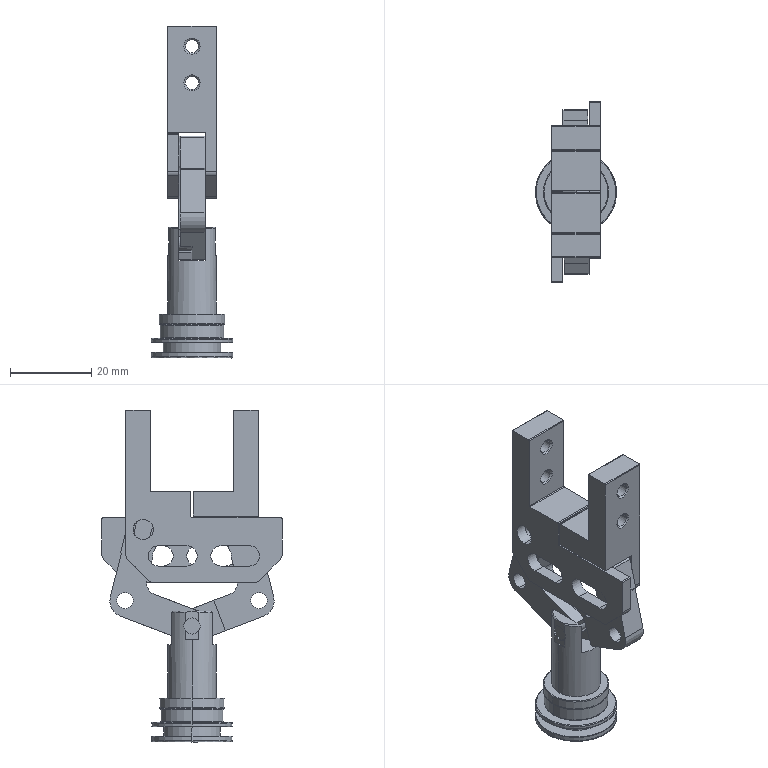Component | SolidWorks | HZ022-HFP20-1_HZ022-HFP20 (1)-1 | 1 solid | 225 faces | volume 14562 mm3 | plane 111 | cylinder 79 | cone 21 | spline 14 | commonest cylinder face diameters 4 x14 5 x12 0.4 x12 3.242 x8 3 x8 1 x5 20 x4 12 x2 | material AL6061